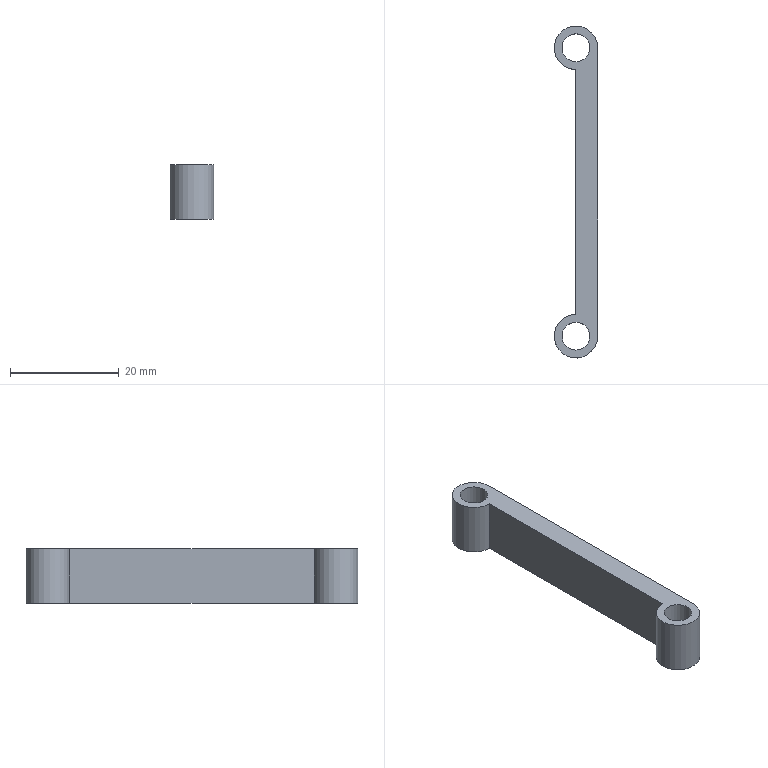Component | NX | PUSH_PLATE | 1 solid | 8 faces | box 8 x 61 x 10 mm | volume 2465 mm3 | cylinder 4 | plane 4 | commonest cylinder face diameters 8 x2 5.1 x2
STEP:
#1=CARTESIAN_POINT('',(0.,0.,0.));
#2=DIRECTION('',(0.,0.,1.));
#3=DIRECTION('',(1.,0.,0.));
#4=AXIS2_PLACEMENT_3D('',#1,#2,#3);
#5=CARTESIAN_POINT('',(-15.538,-20.899,5.633));
#6=VERTEX_POINT('',#5);
#7=CARTESIAN_POINT('',(-11.538,-24.899,5.633));
#8=VERTEX_POINT('',#7);
#9=CARTESIAN_POINT('',(-15.538,-24.899,5.633));
#10=DIRECTION('',(0.,0.,1.));
#11=DIRECTION('',(0.,1.,0.));
#12=AXIS2_PLACEMENT_3D('',#9,#10,#11);
#13=CIRCLE('',#12,4.);
#14=CARTESIAN_POINT('',(-15.538,-24.899,15.633));
#15=DIRECTION('',(0.,0.,-1.));
#16=DIRECTION('',(0.,-1.,0.));
#17=AXIS2_PLACEMENT_3D('',#14,#15,#16);
#18=CYLINDRICAL_SURFACE('',#17,4.);
#19=CARTESIAN_POINT('',(3.142,10.));
#20=DIRECTION('',(-1.,0.));
#21=VECTOR('',#20,1.);
#22=LINE('',#19,#21);
#23=(GEOMETRIC_REPRESENTATION_CONTEXT(2)PARAMETRIC_REPRESENTATION_CONTEXT()REPRESENTATION_CONTEXT('',''));
#24=DEFINITIONAL_REPRESENTATION('',(#22),#23);
#25=PCURVE('',#18,#24);
#26=CARTESIAN_POINT('',(-15.538,-24.899,5.633));
#27=DIRECTION('',(0.,0.,1.));
#28=DIRECTION('',(0.,1.,0.));
#29=AXIS2_PLACEMENT_3D('',#26,#27,#28);
#30=PLANE('',#29);
#31=CARTESIAN_POINT('',(0.,0.));
#32=DIRECTION('',(1.,0.));
#33=AXIS2_PLACEMENT_2D('',#31,#32);
#34=CIRCLE('',#33,4.);
#35=(GEOMETRIC_REPRESENTATION_CONTEXT(2)PARAMETRIC_REPRESENTATION_CONTEXT()REPRESENTATION_CONTEXT('',''));
#36=DEFINITIONAL_REPRESENTATION('',(#34),#35);
#37=PCURVE('',#30,#36);
#38=SURFACE_CURVE('',#13,(#25,#37),.PCURVE_S1.);
#39=EDGE_CURVE('',#6,#8,#38,.T.);
#40=ORIENTED_EDGE('',*,*,#39,.T.);
#41=CARTESIAN_POINT('',(-11.538,-24.899,15.633));
#42=VERTEX_POINT('',#41);
#43=CARTESIAN_POINT('',(-11.538,-24.899,15.633));
#44=DIRECTION('',(0.,0.,-1.));
#45=VECTOR('',#44,1.);
#46=LINE('',#43,#45);
#47=CARTESIAN_POINT('',(-1.571,0.));
#48=DIRECTION('',(0.,1.));
#49=VECTOR('',#48,1.);
#50=LINE('',#47,#49);
#51=(GEOMETRIC_REPRESENTATION_CONTEXT(2)PARAMETRIC_REPRESENTATION_CONTEXT()REPRESENTATION_CONTEXT('',''));
#52=DEFINITIONAL_REPRESENTATION('',(#50),#51);
#53=PCURVE('',#18,#52);
#54=CARTESIAN_POINT('',(-11.538,1.601,15.633));
#55=DIRECTION('',(-1.,-0.,0.));
#56=DIRECTION('',(0.,-1.,0.));
#57=AXIS2_PLACEMENT_3D('',#54,#55,#56);
#58=PLANE('',#57);
#59=CARTESIAN_POINT('',(26.5,0.));
#60=DIRECTION('',(0.,-1.));
#61=VECTOR('',#60,1.);
#62=LINE('',#59,#61);
#63=(GEOMETRIC_REPRESENTATION_CONTEXT(2)PARAMETRIC_REPRESENTATION_CONTEXT()REPRESENTATION_CONTEXT('',''));
#64=DEFINITIONAL_REPRESENTATION('',(#62),#63);
#65=PCURVE('',#58,#64);
#66=SURFACE_CURVE('',#46,(#53,#65),.PCURVE_S1.);
#67=EDGE_CURVE('',#42,#8,#66,.T.);
#68=ORIENTED_EDGE('',*,*,#67,.F.);
#69=CARTESIAN_POINT('',(-15.538,-20.899,15.633));
#70=VERTEX_POINT('',#69);
#71=CARTESIAN_POINT('',(-15.538,-24.899,15.633));
#72=DIRECTION('',(0.,0.,1.));
#73=DIRECTION('',(0.,1.,0.));
#74=AXIS2_PLACEMENT_3D('',#71,#72,#73);
#75=CIRCLE('',#74,4.);
#76=CARTESIAN_POINT('',(3.142,0.));
#77=DIRECTION('',(-1.,0.));
#78=VECTOR('',#77,1.);
#79=LINE('',#76,#78);
#80=(GEOMETRIC_REPRESENTATION_CONTEXT(2)PARAMETRIC_REPRESENTATION_CONTEXT()REPRESENTATION_CONTEXT('',''));
#81=DEFINITIONAL_REPRESENTATION('',(#79),#80);
#82=PCURVE('',#18,#81);
#83=CARTESIAN_POINT('',(-15.538,-24.899,15.633));
#84=DIRECTION('',(0.,0.,1.));
#85=DIRECTION('',(0.,1.,0.));
#86=AXIS2_PLACEMENT_3D('',#83,#84,#85);
#87=PLANE('',#86);
#88=CARTESIAN_POINT('',(0.,0.));
#89=DIRECTION('',(1.,0.));
#90=AXIS2_PLACEMENT_2D('',#88,#89);
#91=CIRCLE('',#90,4.);
#92=(GEOMETRIC_REPRESENTATION_CONTEXT(2)PARAMETRIC_REPRESENTATION_CONTEXT()REPRESENTATION_CONTEXT('',''));
#93=DEFINITIONAL_REPRESENTATION('',(#91),#92);
#94=PCURVE('',#87,#93);
#95=SURFACE_CURVE('',#75,(#82,#94),.PCURVE_S1.);
#96=EDGE_CURVE('',#70,#42,#95,.T.);
#97=ORIENTED_EDGE('',*,*,#96,.F.);
#98=CARTESIAN_POINT('',(-15.538,-20.899,15.633));
#99=DIRECTION('',(0.,0.,-1.));
#100=VECTOR('',#99,1.);
#101=LINE('',#98,#100);
#102=CARTESIAN_POINT('',(3.142,0.));
#103=DIRECTION('',(0.,1.));
#104=VECTOR('',#103,1.);
#105=LINE('',#102,#104);
#106=(GEOMETRIC_REPRESENTATION_CONTEXT(2)PARAMETRIC_REPRESENTATION_CONTEXT()REPRESENTATION_CONTEXT('',''));
#107=DEFINITIONAL_REPRESENTATION('',(#105),#106);
#108=PCURVE('',#18,#107);
#109=CARTESIAN_POINT('',(-15.538,1.601,15.633));
#110=DIRECTION('',(1.,0.,0.));
#111=DIRECTION('',(0.,0.,-1.));
#112=AXIS2_PLACEMENT_3D('',#109,#110,#111);
#113=PLANE('',#112);
#114=CARTESIAN_POINT('',(0.,-22.5));
#115=DIRECTION('',(1.,0.));
#116=VECTOR('',#115,1.);
#117=LINE('',#114,#116);
#118=(GEOMETRIC_REPRESENTATION_CONTEXT(2)PARAMETRIC_REPRESENTATION_CONTEXT()REPRESENTATION_CONTEXT('',''));
#119=DEFINITIONAL_REPRESENTATION('',(#117),#118);
#120=PCURVE('',#113,#119);
#121=SURFACE_CURVE('',#101,(#108,#120),.PCURVE_S1.);
#122=EDGE_CURVE('',#70,#6,#121,.T.);
#123=ORIENTED_EDGE('',*,*,#122,.T.);
#124=EDGE_LOOP('',(#40,#68,#97,#123));
#125=FACE_BOUND('',#124,.T.);
#126=ADVANCED_FACE('',(#125),#18,.T.);
#127=CARTESIAN_POINT('',(-11.538,28.101,5.633));
#128=VERTEX_POINT('',#127);
#129=CARTESIAN_POINT('',(-11.538,1.601,5.633));
#130=DIRECTION('',(-0.,1.,0.));
#131=VECTOR('',#130,1.);
#132=LINE('',#129,#131);
#133=CARTESIAN_POINT('',(0.,-10.));
#134=DIRECTION('',(-1.,0.));
#135=VECTOR('',#134,1.);
#136=LINE('',#133,#135);
#137=(GEOMETRIC_REPRESENTATION_CONTEXT(2)PARAMETRIC_REPRESENTATION_CONTEXT()REPRESENTATION_CONTEXT('',''));
#138=DEFINITIONAL_REPRESENTATION('',(#136),#137);
#139=PCURVE('',#58,#138);
#140=CARTESIAN_POINT('',(26.5,-4.));
#141=DIRECTION('',(1.,0.));
#142=VECTOR('',#141,1.);
#143=LINE('',#140,#142);
#144=(GEOMETRIC_REPRESENTATION_CONTEXT(2)PARAMETRIC_REPRESENTATION_CONTEXT()REPRESENTATION_CONTEXT('',''));
#145=DEFINITIONAL_REPRESENTATION('',(#143),#144);
#146=PCURVE('',#30,#145);
#147=SURFACE_CURVE('',#132,(#139,#146),.PCURVE_S1.);
#148=EDGE_CURVE('',#8,#128,#147,.T.);
#149=ORIENTED_EDGE('',*,*,#148,.T.);
#150=CARTESIAN_POINT('',(-11.538,28.101,15.633));
#151=VERTEX_POINT('',#150);
#152=CARTESIAN_POINT('',(-11.538,28.101,15.633));
#153=DIRECTION('',(0.,0.,-1.));
#154=VECTOR('',#153,1.);
#155=LINE('',#152,#154);
#156=CARTESIAN_POINT('',(-26.5,0.));
#157=DIRECTION('',(0.,-1.));
#158=VECTOR('',#157,1.);
#159=LINE('',#156,#158);
#160=(GEOMETRIC_REPRESENTATION_CONTEXT(2)PARAMETRIC_REPRESENTATION_CONTEXT()REPRESENTATION_CONTEXT('',''));
#161=DEFINITIONAL_REPRESENTATION('',(#159),#160);
#162=PCURVE('',#58,#161);
#163=CARTESIAN_POINT('',(-15.538,28.101,15.633));
#164=DIRECTION('',(0.,0.,-1.));
#165=DIRECTION('',(0.,-1.,0.));
#166=AXIS2_PLACEMENT_3D('',#163,#164,#165);
#167=CYLINDRICAL_SURFACE('',#166,4.);
#168=CARTESIAN_POINT('',(4.712,0.));
#169=DIRECTION('',(0.,1.));
#170=VECTOR('',#169,1.);
#171=LINE('',#168,#170);
#172=(GEOMETRIC_REPRESENTATION_CONTEXT(2)PARAMETRIC_REPRESENTATION_CONTEXT()REPRESENTATION_CONTEXT('',''));
#173=DEFINITIONAL_REPRESENTATION('',(#171),#172);
#174=PCURVE('',#167,#173);
#175=SURFACE_CURVE('',#155,(#162,#174),.PCURVE_S1.);
#176=EDGE_CURVE('',#151,#128,#175,.T.);
#177=ORIENTED_EDGE('',*,*,#176,.F.);
#178=CARTESIAN_POINT('',(-11.538,-24.899,15.633));
#179=DIRECTION('',(-0.,1.,0.));
#180=VECTOR('',#179,1.);
#181=LINE('',#178,#180);
#182=CARTESIAN_POINT('',(26.5,0.));
#183=DIRECTION('',(-1.,0.));
#184=VECTOR('',#183,1.);
#185=LINE('',#182,#184);
#186=(GEOMETRIC_REPRESENTATION_CONTEXT(2)PARAMETRIC_REPRESENTATION_CONTEXT()REPRESENTATION_CONTEXT('',''));
#187=DEFINITIONAL_REPRESENTATION('',(#185),#186);
#188=PCURVE('',#58,#187);
#189=CARTESIAN_POINT('',(0.,-4.));
#190=DIRECTION('',(1.,0.));
#191=VECTOR('',#190,1.);
#192=LINE('',#189,#191);
#193=(GEOMETRIC_REPRESENTATION_CONTEXT(2)PARAMETRIC_REPRESENTATION_CONTEXT()REPRESENTATION_CONTEXT('',''));
#194=DEFINITIONAL_REPRESENTATION('',(#192),#193);
#195=PCURVE('',#87,#194);
#196=SURFACE_CURVE('',#181,(#188,#195),.PCURVE_S1.);
#197=EDGE_CURVE('',#42,#151,#196,.T.);
#198=ORIENTED_EDGE('',*,*,#197,.F.);
#199=ORIENTED_EDGE('',*,*,#67,.T.);
#200=EDGE_LOOP('',(#149,#177,#198,#199));
#201=FACE_BOUND('',#200,.T.);
#202=ADVANCED_FACE('',(#201),#58,.F.);
#203=CARTESIAN_POINT('',(-15.538,24.101,5.633));
#204=VERTEX_POINT('',#203);
#205=CARTESIAN_POINT('',(-15.538,28.101,5.633));
#206=DIRECTION('',(0.,0.,1.));
#207=DIRECTION('',(0.,-1.,0.));
#208=AXIS2_PLACEMENT_3D('',#205,#206,#207);
#209=CIRCLE('',#208,4.);
#210=CARTESIAN_POINT('',(6.283,10.));
#211=DIRECTION('',(-1.,0.));
#212=VECTOR('',#211,1.);
#213=LINE('',#210,#212);
#214=(GEOMETRIC_REPRESENTATION_CONTEXT(2)PARAMETRIC_REPRESENTATION_CONTEXT()REPRESENTATION_CONTEXT('',''));
#215=DEFINITIONAL_REPRESENTATION('',(#213),#214);
#216=PCURVE('',#167,#215);
#217=CARTESIAN_POINT('',(53.,0.));
#218=DIRECTION('',(-1.,0.));
#219=AXIS2_PLACEMENT_2D('',#217,#218);
#220=CIRCLE('',#219,4.);
#221=(GEOMETRIC_REPRESENTATION_CONTEXT(2)PARAMETRIC_REPRESENTATION_CONTEXT()REPRESENTATION_CONTEXT('',''));
#222=DEFINITIONAL_REPRESENTATION('',(#220),#221);
#223=PCURVE('',#30,#222);
#224=SURFACE_CURVE('',#209,(#216,#223),.PCURVE_S1.);
#225=EDGE_CURVE('',#128,#204,#224,.T.);
#226=ORIENTED_EDGE('',*,*,#225,.T.);
#227=CARTESIAN_POINT('',(-15.538,24.101,15.633));
#228=VERTEX_POINT('',#227);
#229=CARTESIAN_POINT('',(-15.538,24.101,15.633));
#230=DIRECTION('',(0.,0.,-1.));
#231=VECTOR('',#230,1.);
#232=LINE('',#229,#231);
#233=CARTESIAN_POINT('',(0.,0.));
#234=DIRECTION('',(0.,1.));
#235=VECTOR('',#234,1.);
#236=LINE('',#233,#235);
#237=(GEOMETRIC_REPRESENTATION_CONTEXT(2)PARAMETRIC_REPRESENTATION_CONTEXT()REPRESENTATION_CONTEXT('',''));
#238=DEFINITIONAL_REPRESENTATION('',(#236),#237);
#239=PCURVE('',#167,#238);
#240=CARTESIAN_POINT('',(0.,22.5));
#241=DIRECTION('',(1.,0.));
#242=VECTOR('',#241,1.);
#243=LINE('',#240,#242);
#244=(GEOMETRIC_REPRESENTATION_CONTEXT(2)PARAMETRIC_REPRESENTATION_CONTEXT()REPRESENTATION_CONTEXT('',''));
#245=DEFINITIONAL_REPRESENTATION('',(#243),#244);
#246=PCURVE('',#113,#245);
#247=SURFACE_CURVE('',#232,(#239,#246),.PCURVE_S1.);
#248=EDGE_CURVE('',#228,#204,#247,.T.);
#249=ORIENTED_EDGE('',*,*,#248,.F.);
#250=CARTESIAN_POINT('',(-15.538,28.101,15.633));
#251=DIRECTION('',(0.,0.,1.));
#252=DIRECTION('',(0.,-1.,0.));
#253=AXIS2_PLACEMENT_3D('',#250,#251,#252);
#254=CIRCLE('',#253,4.);
#255=CARTESIAN_POINT('',(6.283,0.));
#256=DIRECTION('',(-1.,0.));
#257=VECTOR('',#256,1.);
#258=LINE('',#255,#257);
#259=(GEOMETRIC_REPRESENTATION_CONTEXT(2)PARAMETRIC_REPRESENTATION_CONTEXT()REPRESENTATION_CONTEXT('',''));
#260=DEFINITIONAL_REPRESENTATION('',(#258),#259);
#261=PCURVE('',#167,#260);
#262=CARTESIAN_POINT('',(53.,0.));
#263=DIRECTION('',(-1.,0.));
#264=AXIS2_PLACEMENT_2D('',#262,#263);
#265=CIRCLE('',#264,4.);
#266=(GEOMETRIC_REPRESENTATION_CONTEXT(2)PARAMETRIC_REPRESENTATION_CONTEXT()REPRESENTATION_CONTEXT('',''));
#267=DEFINITIONAL_REPRESENTATION('',(#265),#266);
#268=PCURVE('',#87,#267);
#269=SURFACE_CURVE('',#254,(#261,#268),.PCURVE_S1.);
#270=EDGE_CURVE('',#151,#228,#269,.T.);
#271=ORIENTED_EDGE('',*,*,#270,.F.);
#272=ORIENTED_EDGE('',*,*,#176,.T.);
#273=EDGE_LOOP('',(#226,#249,#271,#272));
#274=FACE_BOUND('',#273,.T.);
#275=ADVANCED_FACE('',(#274),#167,.T.);
#276=CARTESIAN_POINT('',(-15.538,-27.449,15.633));
#277=VERTEX_POINT('',#276);
#278=CARTESIAN_POINT('',(-15.538,-24.899,15.633));
#279=DIRECTION('',(0.,0.,-1.));
#280=DIRECTION('',(0.,-1.,0.));
#281=AXIS2_PLACEMENT_3D('',#278,#279,#280);
#282=CIRCLE('',#281,2.55);
#283=CARTESIAN_POINT('',(-15.538,-24.899,15.633));
#284=DIRECTION('',(0.,0.,-1.));
#285=DIRECTION('',(0.,-1.,0.));
#286=AXIS2_PLACEMENT_3D('',#283,#284,#285);
#287=CYLINDRICAL_SURFACE('',#286,2.55);
#288=CARTESIAN_POINT('',(0.,0.));
#289=DIRECTION('',(1.,0.));
#290=VECTOR('',#289,1.);
#291=LINE('',#288,#290);
#292=(GEOMETRIC_REPRESENTATION_CONTEXT(2)PARAMETRIC_REPRESENTATION_CONTEXT()REPRESENTATION_CONTEXT('',''));
#293=DEFINITIONAL_REPRESENTATION('',(#291),#292);
#294=PCURVE('',#287,#293);
#295=CARTESIAN_POINT('',(-2.55,0.));
#296=CARTESIAN_POINT('',(-2.55,4.417));
#297=CARTESIAN_POINT('',(1.275,2.208));
#298=CARTESIAN_POINT('',(5.1,0.));
#299=CARTESIAN_POINT('',(1.275,-2.208));
#300=CARTESIAN_POINT('',(-2.55,-4.417));
#301=CARTESIAN_POINT('',(-2.55,0.));
#302=(BOUNDED_CURVE()B_SPLINE_CURVE(2,(#295,#296,#297,#298,#299,#300,#301),.UNSPECIFIED.,.T.,.F.)B_SPLINE_CURVE_WITH_KNOTS((1,2,2,2,2,1),(-2.094,0.,2.094,4.189,6.283,8.378),.UNSPECIFIED.)CURVE()GEOMETRIC_REPRESENTATION_ITEM()RATIONAL_B_SPLINE_CURVE((1.,0.5,1.,0.5,1.,0.5,1.))REPRESENTATION_ITEM(''));
#303=(GEOMETRIC_REPRESENTATION_CONTEXT(2)PARAMETRIC_REPRESENTATION_CONTEXT()REPRESENTATION_CONTEXT('',''));
#304=DEFINITIONAL_REPRESENTATION('',(#302),#303);
#305=PCURVE('',#87,#304);
#306=SURFACE_CURVE('',#282,(#294,#305),.PCURVE_S1.);
#307=EDGE_CURVE('',#277,#277,#306,.T.);
#308=ORIENTED_EDGE('',*,*,#307,.T.);
#309=CARTESIAN_POINT('',(-15.538,-27.449,5.633));
#310=VERTEX_POINT('',#309);
#311=CARTESIAN_POINT('',(-15.538,-27.449,15.633));
#312=CARTESIAN_POINT('',(-15.538,-27.449,5.633));
#313=B_SPLINE_CURVE_WITH_KNOTS('',1,(#311,#312),.UNSPECIFIED.,.F.,.F.,(2,2),(0.,10.),.PIECEWISE_BEZIER_KNOTS.);
#314=CARTESIAN_POINT('',(6.283,0.));
#315=DIRECTION('',(0.,1.));
#316=VECTOR('',#315,1.);
#317=LINE('',#314,#316);
#318=(GEOMETRIC_REPRESENTATION_CONTEXT(2)PARAMETRIC_REPRESENTATION_CONTEXT()REPRESENTATION_CONTEXT('',''));
#319=DEFINITIONAL_REPRESENTATION('',(#317),#318);
#320=PCURVE('',#287,#319);
#321=CARTESIAN_POINT('',(0.,0.));
#322=DIRECTION('',(0.,1.));
#323=VECTOR('',#322,1.);
#324=LINE('',#321,#323);
#325=(GEOMETRIC_REPRESENTATION_CONTEXT(2)PARAMETRIC_REPRESENTATION_CONTEXT()REPRESENTATION_CONTEXT('',''));
#326=DEFINITIONAL_REPRESENTATION('',(#324),#325);
#327=PCURVE('',#287,#326);
#328=SEAM_CURVE('',#313,(#320,#327),.PCURVE_S1.);
#329=EDGE_CURVE('',#277,#310,#328,.T.);
#330=ORIENTED_EDGE('',*,*,#329,.T.);
#331=CARTESIAN_POINT('',(-15.538,-24.899,5.633));
#332=DIRECTION('',(0.,0.,-1.));
#333=DIRECTION('',(0.,-1.,0.));
#334=AXIS2_PLACEMENT_3D('',#331,#332,#333);
#335=CIRCLE('',#334,2.55);
#336=CARTESIAN_POINT('',(0.,10.));
#337=DIRECTION('',(1.,0.));
#338=VECTOR('',#337,1.);
#339=LINE('',#336,#338);
#340=(GEOMETRIC_REPRESENTATION_CONTEXT(2)PARAMETRIC_REPRESENTATION_CONTEXT()REPRESENTATION_CONTEXT('',''));
#341=DEFINITIONAL_REPRESENTATION('',(#339),#340);
#342=PCURVE('',#287,#341);
#343=CARTESIAN_POINT('',(-2.55,0.));
#344=CARTESIAN_POINT('',(-2.55,4.417));
#345=CARTESIAN_POINT('',(1.275,2.208));
#346=CARTESIAN_POINT('',(5.1,0.));
#347=CARTESIAN_POINT('',(1.275,-2.208));
#348=CARTESIAN_POINT('',(-2.55,-4.417));
#349=CARTESIAN_POINT('',(-2.55,0.));
#350=(BOUNDED_CURVE()B_SPLINE_CURVE(2,(#343,#344,#345,#346,#347,#348,#349),.UNSPECIFIED.,.T.,.F.)B_SPLINE_CURVE_WITH_KNOTS((1,2,2,2,2,1),(-2.094,0.,2.094,4.189,6.283,8.378),.UNSPECIFIED.)CURVE()GEOMETRIC_REPRESENTATION_ITEM()RATIONAL_B_SPLINE_CURVE((1.,0.5,1.,0.5,1.,0.5,1.))REPRESENTATION_ITEM(''));
#351=(GEOMETRIC_REPRESENTATION_CONTEXT(2)PARAMETRIC_REPRESENTATION_CONTEXT()REPRESENTATION_CONTEXT('',''));
#352=DEFINITIONAL_REPRESENTATION('',(#350),#351);
#353=PCURVE('',#30,#352);
#354=SURFACE_CURVE('',#335,(#342,#353),.PCURVE_S1.);
#355=EDGE_CURVE('',#310,#310,#354,.T.);
#356=ORIENTED_EDGE('',*,*,#355,.F.);
#357=ORIENTED_EDGE('',*,*,#329,.F.);
#358=EDGE_LOOP('',(#308,#330,#356,#357));
#359=FACE_BOUND('',#358,.F.);
#360=ADVANCED_FACE('',(#359),#287,.F.);
#361=CARTESIAN_POINT('',(-15.538,1.601,5.633));
#362=DIRECTION('',(0.,-1.,0.));
#363=VECTOR('',#362,1.);
#364=LINE('',#361,#363);
#365=CARTESIAN_POINT('',(10.,0.));
#366=DIRECTION('',(0.,-1.));
#367=VECTOR('',#366,1.);
#368=LINE('',#365,#367);
#369=(GEOMETRIC_REPRESENTATION_CONTEXT(2)PARAMETRIC_REPRESENTATION_CONTEXT()REPRESENTATION_CONTEXT('',''));
#370=DEFINITIONAL_REPRESENTATION('',(#368),#369);
#371=PCURVE('',#113,#370);
#372=CARTESIAN_POINT('',(26.5,0.));
#373=DIRECTION('',(-1.,0.));
#374=VECTOR('',#373,1.);
#375=LINE('',#372,#374);
#376=(GEOMETRIC_REPRESENTATION_CONTEXT(2)PARAMETRIC_REPRESENTATION_CONTEXT()REPRESENTATION_CONTEXT('',''));
#377=DEFINITIONAL_REPRESENTATION('',(#375),#376);
#378=PCURVE('',#30,#377);
#379=SURFACE_CURVE('',#364,(#371,#378),.PCURVE_S1.);
#380=EDGE_CURVE('',#204,#6,#379,.T.);
#381=ORIENTED_EDGE('',*,*,#380,.T.);
#382=ORIENTED_EDGE('',*,*,#122,.F.);
#383=CARTESIAN_POINT('',(-15.538,24.101,15.633));
#384=DIRECTION('',(0.,-1.,0.));
#385=VECTOR('',#384,1.);
#386=LINE('',#383,#385);
#387=CARTESIAN_POINT('',(0.,22.5));
#388=DIRECTION('',(0.,-1.));
#389=VECTOR('',#388,1.);
#390=LINE('',#387,#389);
#391=(GEOMETRIC_REPRESENTATION_CONTEXT(2)PARAMETRIC_REPRESENTATION_CONTEXT()REPRESENTATION_CONTEXT('',''));
#392=DEFINITIONAL_REPRESENTATION('',(#390),#391);
#393=PCURVE('',#113,#392);
#394=CARTESIAN_POINT('',(49.,0.));
#395=DIRECTION('',(-1.,-0.));
#396=VECTOR('',#395,1.);
#397=LINE('',#394,#396);
#398=(GEOMETRIC_REPRESENTATION_CONTEXT(2)PARAMETRIC_REPRESENTATION_CONTEXT()REPRESENTATION_CONTEXT('',''));
#399=DEFINITIONAL_REPRESENTATION('',(#397),#398);
#400=PCURVE('',#87,#399);
#401=SURFACE_CURVE('',#386,(#393,#400),.PCURVE_S1.);
#402=EDGE_CURVE('',#228,#70,#401,.T.);
#403=ORIENTED_EDGE('',*,*,#402,.F.);
#404=ORIENTED_EDGE('',*,*,#248,.T.);
#405=EDGE_LOOP('',(#381,#382,#403,#404));
#406=FACE_BOUND('',#405,.T.);
#407=ADVANCED_FACE('',(#406),#113,.F.);
#408=CARTESIAN_POINT('',(-15.538,30.651,15.633));
#409=VERTEX_POINT('',#408);
#410=CARTESIAN_POINT('',(-15.538,28.101,15.633));
#411=DIRECTION('',(0.,0.,1.));
#412=DIRECTION('',(0.,1.,0.));
#413=AXIS2_PLACEMENT_3D('',#410,#411,#412);
#414=CIRCLE('',#413,2.55);
#415=CARTESIAN_POINT('',(-15.538,28.101,15.633));
#416=DIRECTION('',(0.,0.,-1.));
#417=DIRECTION('',(0.,-1.,0.));
#418=AXIS2_PLACEMENT_3D('',#415,#416,#417);
#419=CYLINDRICAL_SURFACE('',#418,2.55);
#420=CARTESIAN_POINT('',(9.425,0.));
#421=DIRECTION('',(-1.,0.));
#422=VECTOR('',#421,1.);
#423=LINE('',#420,#422);
#424=(GEOMETRIC_REPRESENTATION_CONTEXT(2)PARAMETRIC_REPRESENTATION_CONTEXT()REPRESENTATION_CONTEXT('',''));
#425=DEFINITIONAL_REPRESENTATION('',(#423),#424);
#426=PCURVE('',#419,#425);
#427=CARTESIAN_POINT('',(53.,0.));
#428=DIRECTION('',(1.,0.));
#429=AXIS2_PLACEMENT_2D('',#427,#428);
#430=CIRCLE('',#429,2.55);
#431=(GEOMETRIC_REPRESENTATION_CONTEXT(2)PARAMETRIC_REPRESENTATION_CONTEXT()REPRESENTATION_CONTEXT('',''));
#432=DEFINITIONAL_REPRESENTATION('',(#430),#431);
#433=PCURVE('',#87,#432);
#434=SURFACE_CURVE('',#414,(#426,#433),.PCURVE_S1.);
#435=EDGE_CURVE('',#409,#409,#434,.T.);
#436=ORIENTED_EDGE('',*,*,#435,.F.);
#437=CARTESIAN_POINT('',(-15.538,30.651,5.633));
#438=VERTEX_POINT('',#437);
#439=CARTESIAN_POINT('',(-15.538,30.651,15.633));
#440=CARTESIAN_POINT('',(-15.538,30.651,5.633));
#441=B_SPLINE_CURVE_WITH_KNOTS('',1,(#439,#440),.UNSPECIFIED.,.F.,.F.,(2,2),(0.,10.),.PIECEWISE_BEZIER_KNOTS.);
#442=CARTESIAN_POINT('',(9.425,0.));
#443=DIRECTION('',(0.,1.));
#444=VECTOR('',#443,1.);
#445=LINE('',#442,#444);
#446=(GEOMETRIC_REPRESENTATION_CONTEXT(2)PARAMETRIC_REPRESENTATION_CONTEXT()REPRESENTATION_CONTEXT('',''));
#447=DEFINITIONAL_REPRESENTATION('',(#445),#446);
#448=PCURVE('',#419,#447);
#449=CARTESIAN_POINT('',(3.142,0.));
#450=DIRECTION('',(0.,1.));
#451=VECTOR('',#450,1.);
#452=LINE('',#449,#451);
#453=(GEOMETRIC_REPRESENTATION_CONTEXT(2)PARAMETRIC_REPRESENTATION_CONTEXT()REPRESENTATION_CONTEXT('',''));
#454=DEFINITIONAL_REPRESENTATION('',(#452),#453);
#455=PCURVE('',#419,#454);
#456=SEAM_CURVE('',#441,(#448,#455),.PCURVE_S1.);
#457=EDGE_CURVE('',#409,#438,#456,.T.);
#458=ORIENTED_EDGE('',*,*,#457,.T.);
#459=CARTESIAN_POINT('',(-15.538,28.101,5.633));
#460=DIRECTION('',(0.,0.,1.));
#461=DIRECTION('',(0.,1.,0.));
#462=AXIS2_PLACEMENT_3D('',#459,#460,#461);
#463=CIRCLE('',#462,2.55);
#464=CARTESIAN_POINT('',(9.425,10.));
#465=DIRECTION('',(-1.,0.));
#466=VECTOR('',#465,1.);
#467=LINE('',#464,#466);
#468=(GEOMETRIC_REPRESENTATION_CONTEXT(2)PARAMETRIC_REPRESENTATION_CONTEXT()REPRESENTATION_CONTEXT('',''));
#469=DEFINITIONAL_REPRESENTATION('',(#467),#468);
#470=PCURVE('',#419,#469);
#471=CARTESIAN_POINT('',(53.,0.));
#472=DIRECTION('',(1.,0.));
#473=AXIS2_PLACEMENT_2D('',#471,#472);
#474=CIRCLE('',#473,2.55);
#475=(GEOMETRIC_REPRESENTATION_CONTEXT(2)PARAMETRIC_REPRESENTATION_CONTEXT()REPRESENTATION_CONTEXT('',''));
#476=DEFINITIONAL_REPRESENTATION('',(#474),#475);
#477=PCURVE('',#30,#476);
#478=SURFACE_CURVE('',#463,(#470,#477),.PCURVE_S1.);
#479=EDGE_CURVE('',#438,#438,#478,.T.);
#480=ORIENTED_EDGE('',*,*,#479,.T.);
#481=ORIENTED_EDGE('',*,*,#457,.F.);
#482=EDGE_LOOP('',(#436,#458,#480,#481));
#483=FACE_BOUND('',#482,.F.);
#484=ADVANCED_FACE('',(#483),#419,.F.);
#485=ORIENTED_EDGE('',*,*,#96,.T.);
#486=ORIENTED_EDGE('',*,*,#197,.T.);
#487=ORIENTED_EDGE('',*,*,#270,.T.);
#488=ORIENTED_EDGE('',*,*,#402,.T.);
#489=EDGE_LOOP('',(#485,#486,#487,#488));
#490=FACE_BOUND('',#489,.T.);
#491=ORIENTED_EDGE('',*,*,#307,.T.);
#492=EDGE_LOOP('',(#491));
#493=FACE_BOUND('',#492,.T.);
#494=ORIENTED_EDGE('',*,*,#435,.F.);
#495=EDGE_LOOP('',(#494));
#496=FACE_BOUND('',#495,.T.);
#497=ADVANCED_FACE('',(#490,#493,#496),#87,.T.);
#498=ORIENTED_EDGE('',*,*,#39,.F.);
#499=ORIENTED_EDGE('',*,*,#380,.F.);
#500=ORIENTED_EDGE('',*,*,#225,.F.);
#501=ORIENTED_EDGE('',*,*,#148,.F.);
#502=EDGE_LOOP('',(#498,#499,#500,#501));
#503=FACE_BOUND('',#502,.T.);
#504=ORIENTED_EDGE('',*,*,#355,.F.);
#505=EDGE_LOOP('',(#504));
#506=FACE_BOUND('',#505,.T.);
#507=ORIENTED_EDGE('',*,*,#479,.T.);
#508=EDGE_LOOP('',(#507));
#509=FACE_BOUND('',#508,.T.);
#510=ADVANCED_FACE('',(#503,#506,#509),#30,.F.);
#511=CLOSED_SHELL('',(#126,#202,#275,#360,#407,#484,#497,#510));
#512=MANIFOLD_SOLID_BREP('',#511);
#513=(LENGTH_UNIT()NAMED_UNIT(*)SI_UNIT(.MILLI.,.METRE.));
#514=UNCERTAINTY_MEASURE_WITH_UNIT(LENGTH_MEASURE(0.000002),#513,'','');
#515=(NAMED_UNIT(*)PLANE_ANGLE_UNIT()SI_UNIT($,.RADIAN.));
#516=(NAMED_UNIT(*)SI_UNIT($,.STERADIAN.)SOLID_ANGLE_UNIT());
#517=(GEOMETRIC_REPRESENTATION_CONTEXT(3)GLOBAL_UNCERTAINTY_ASSIGNED_CONTEXT((#514))GLOBAL_UNIT_ASSIGNED_CONTEXT((#513,#515,#516))REPRESENTATION_CONTEXT('',''));
#518=ADVANCED_BREP_SHAPE_REPRESENTATION('',(#4,#512),#517);